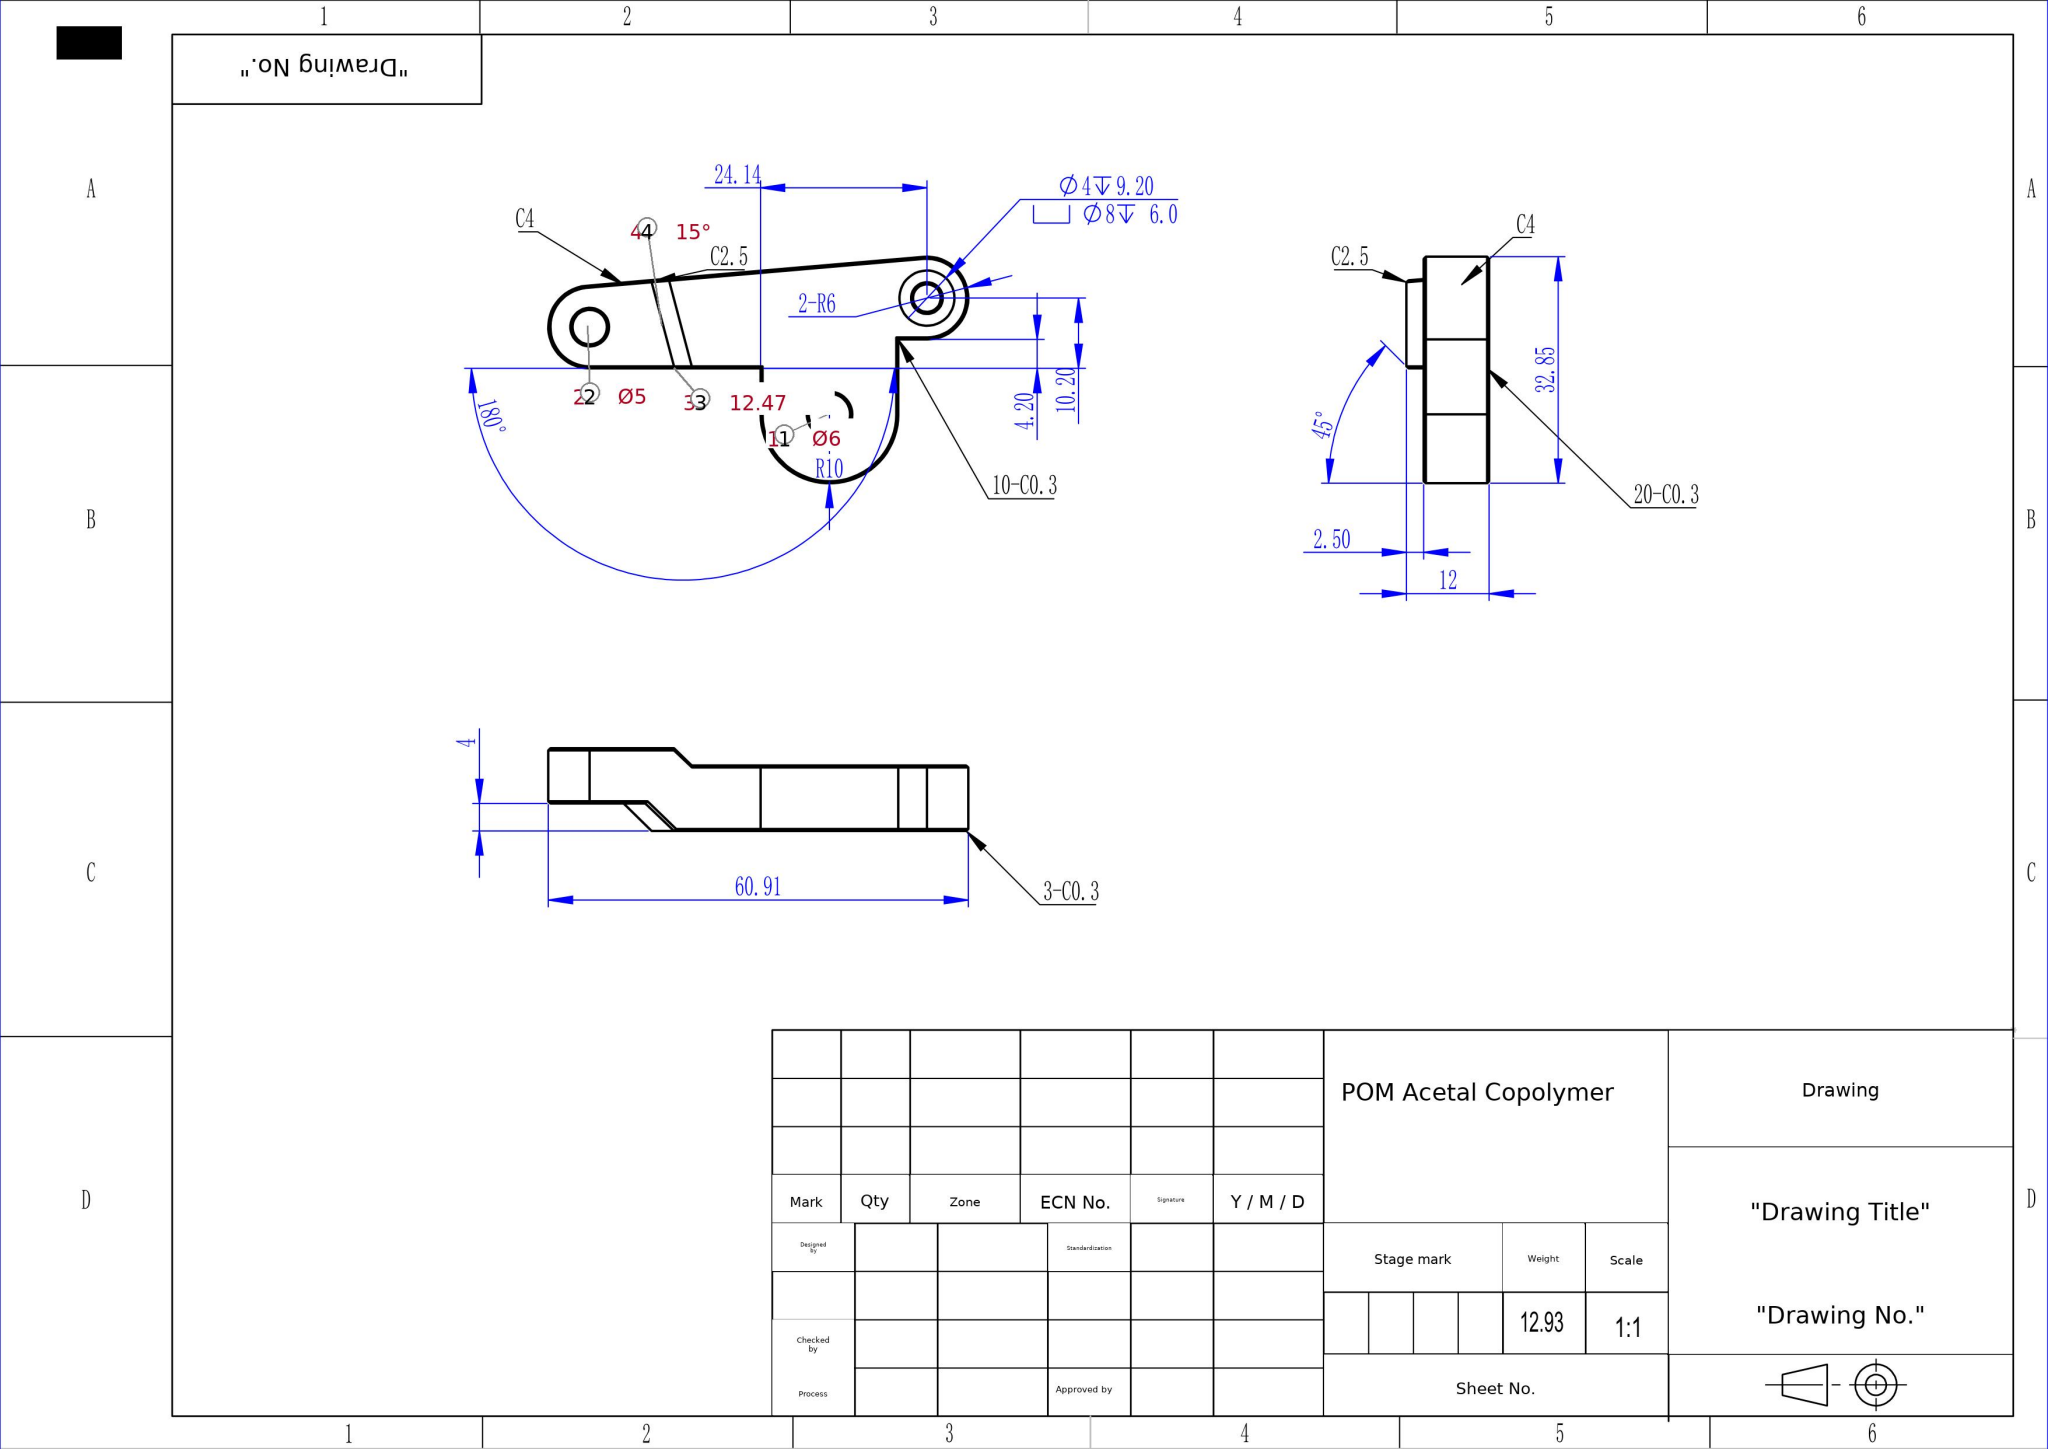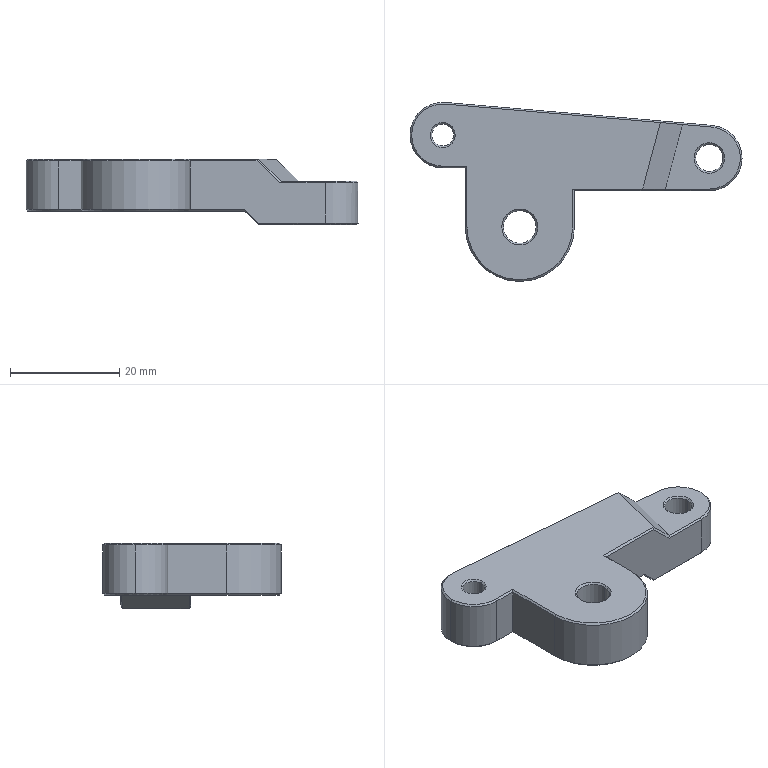Part | SolidWorks | mm | material POM Acetal Copolymer | 1 solid | 62 faces | box 60.91 x 32.85 x 12 mm | volume 9300 mm3 | plane 30 | cone 20 | cylinder 12 | commonest cylinder face diameters 12 x3 8 x2 5 x2 6 x2 4 x2 20 x1